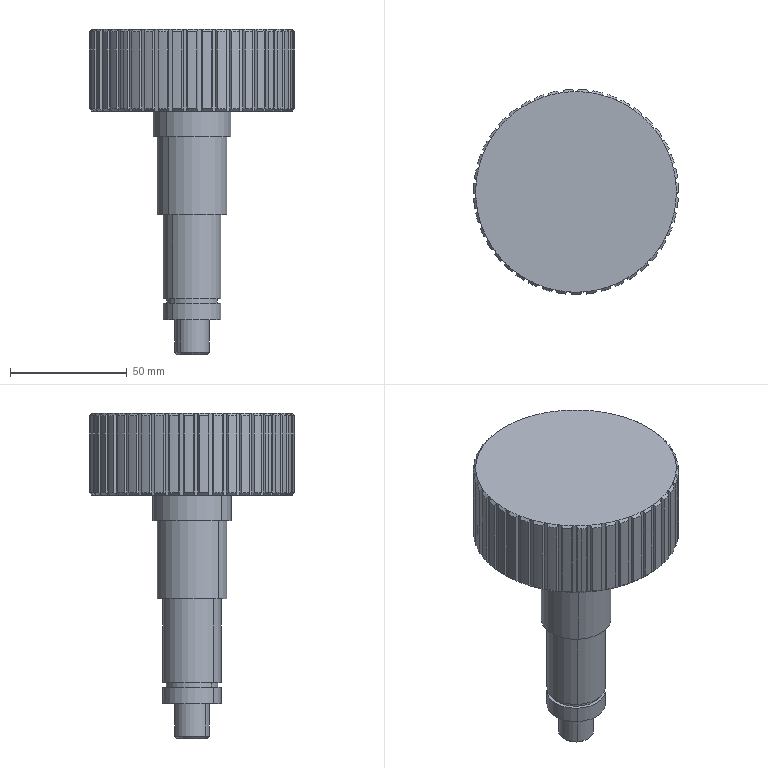Component | SolidWorks | 12AEncoderWheel-1_12AEncoderAxis-1 | 1 solid | 282 faces | volume 267554 mm3 | cylinder 99 | plane 94 | cone 89 | commonest cylinder face diameters 88 x44 86 x43 25 x4 15 x2 22 x2 30 x2 33.5 x2